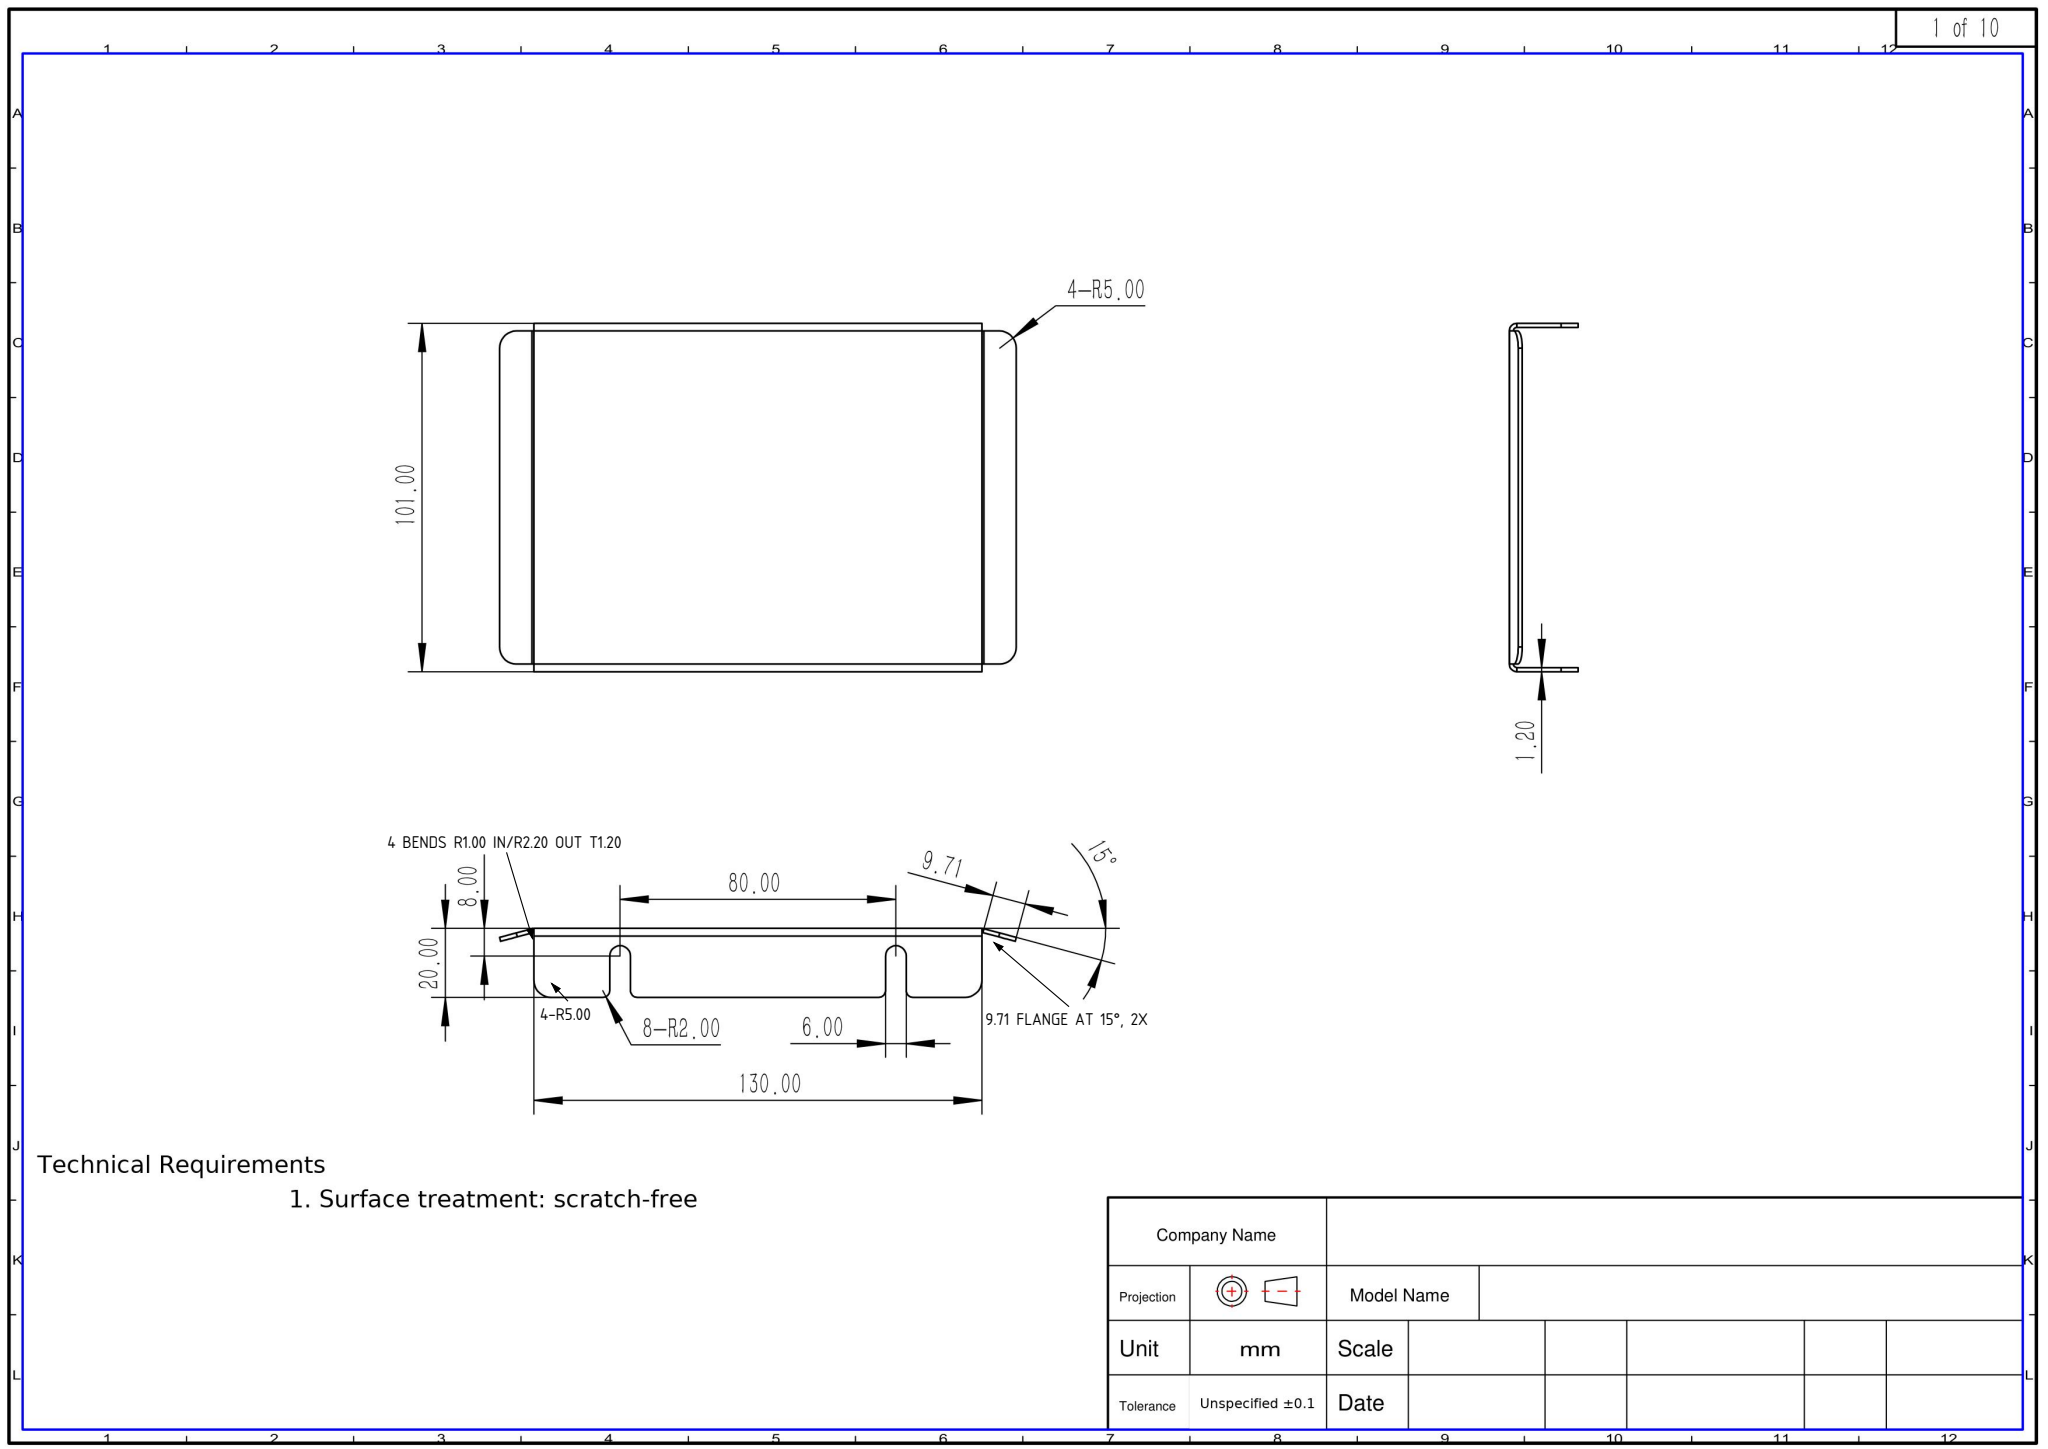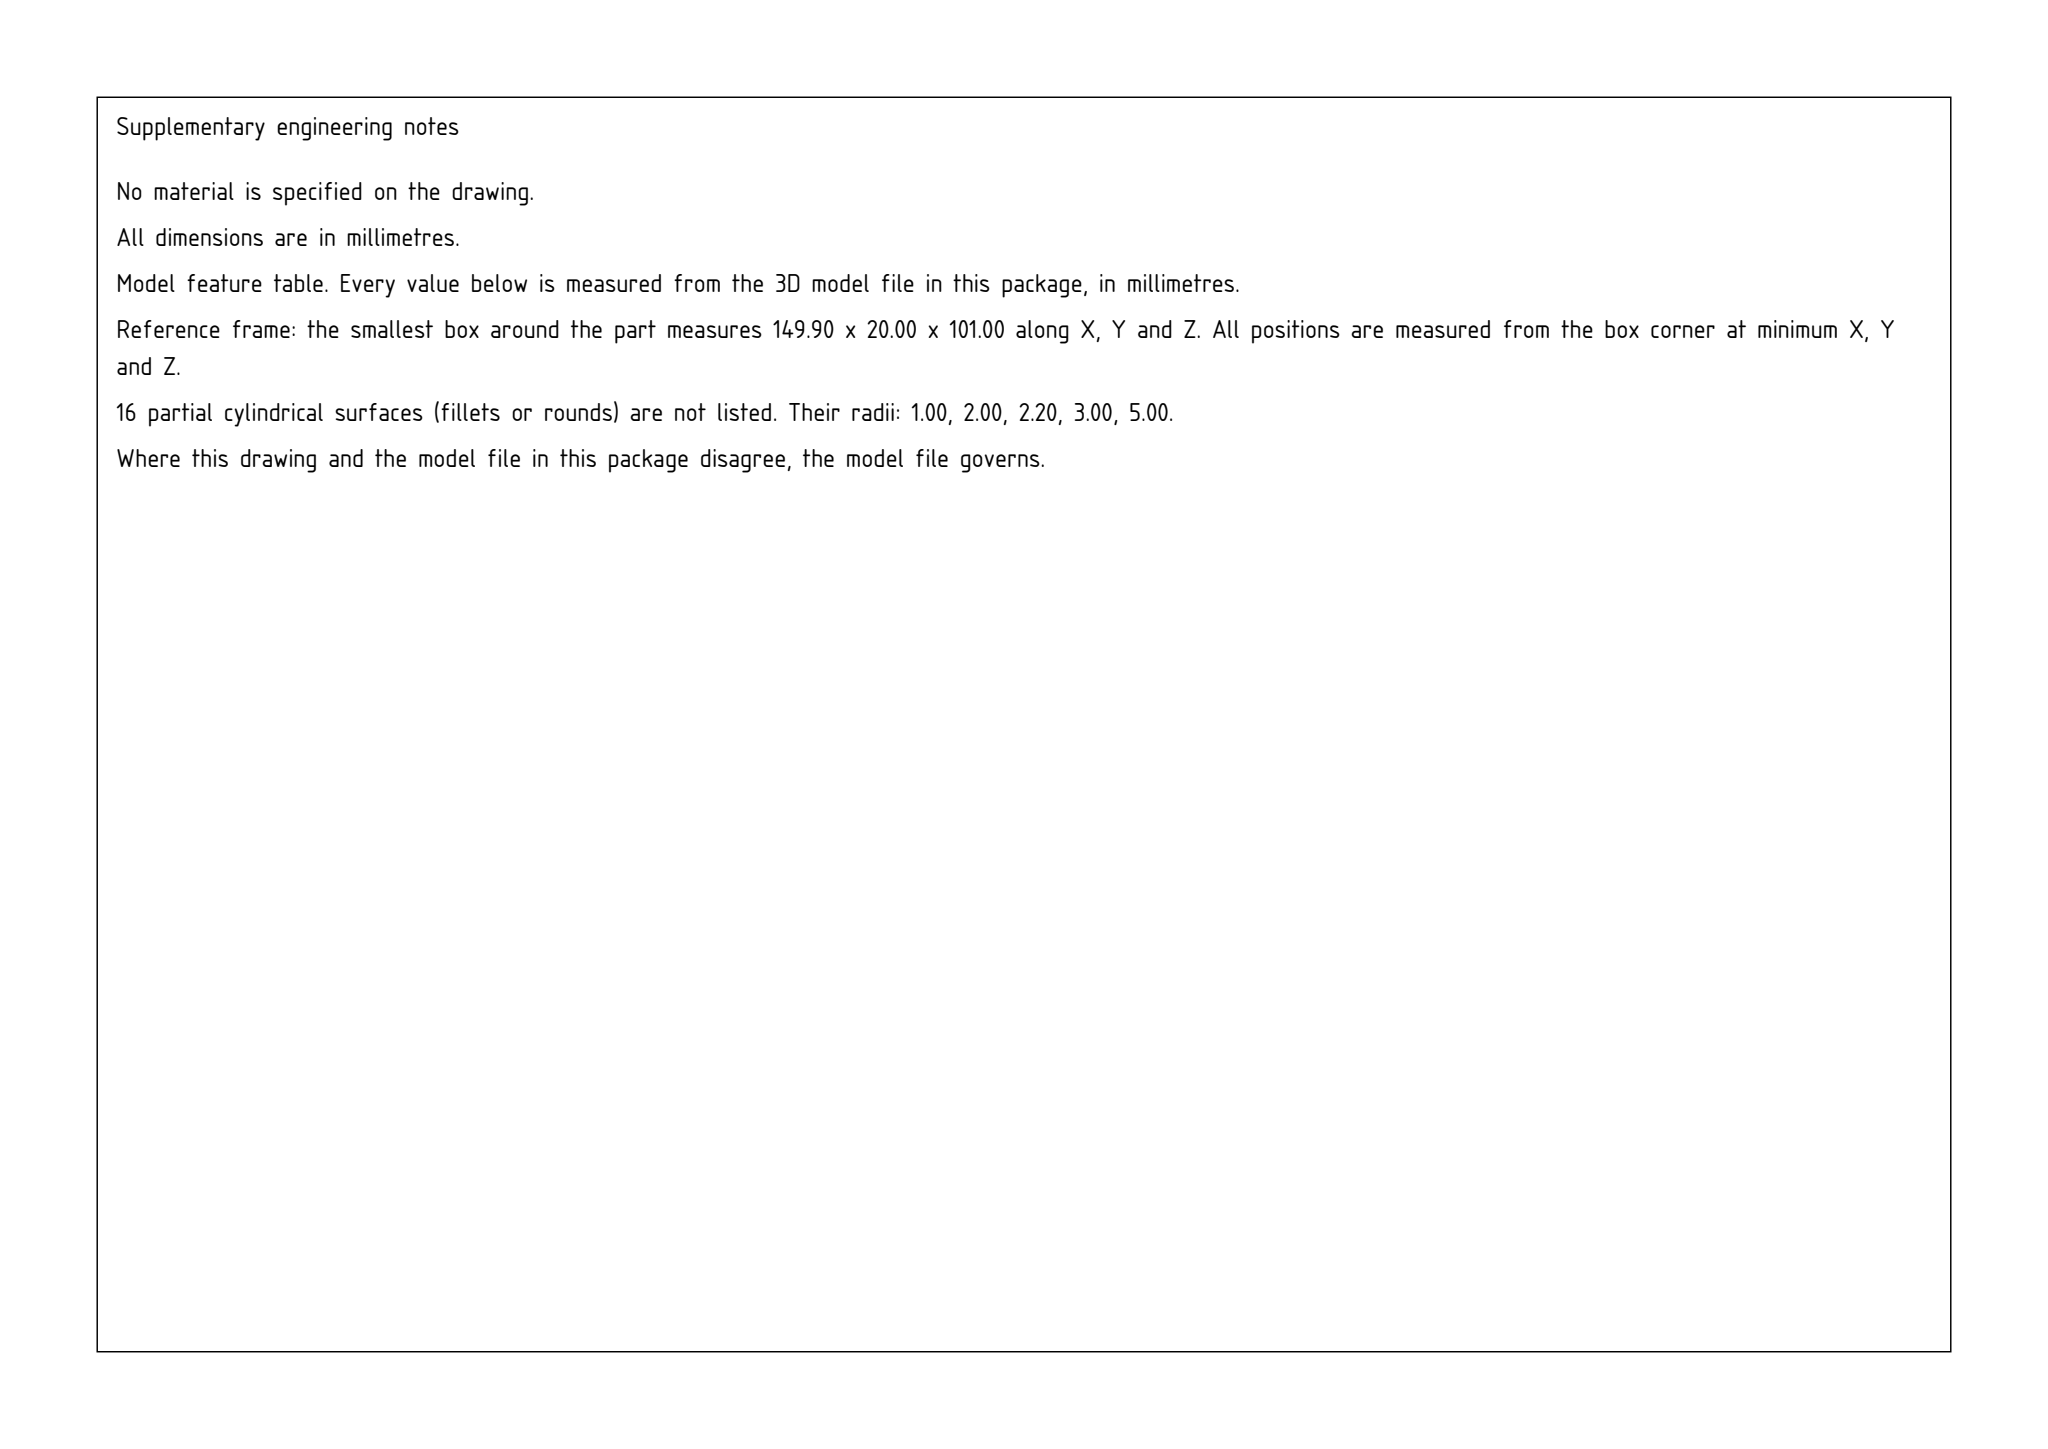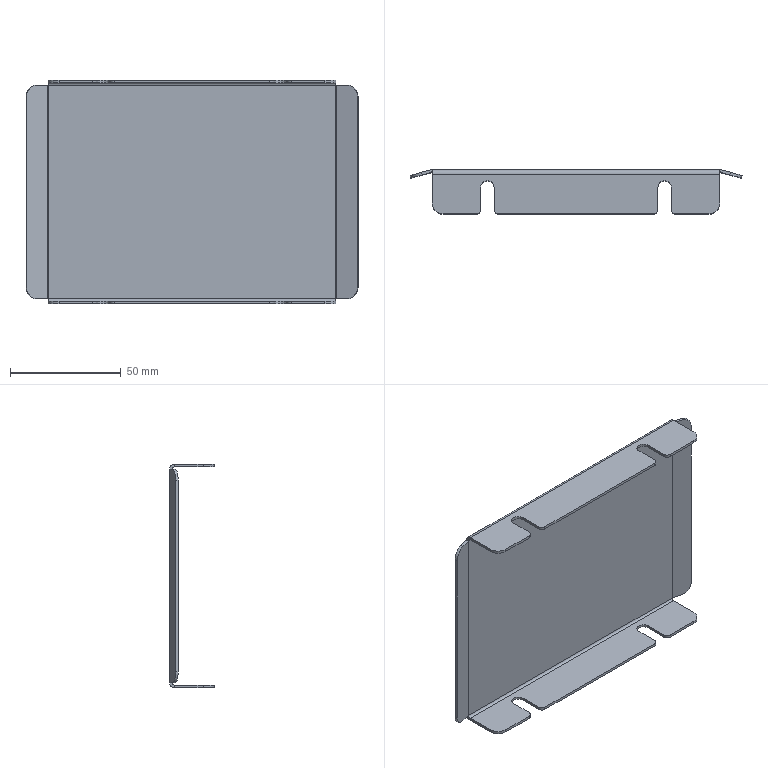Part | SolidWorks | mm | 1 solid | 70 faces | box 149.9 x 20 x 101 mm | volume 23283 mm3 | plane 42 | cylinder 28 | commonest cylinder face diameters 10 x8 4 x8 4.4 x4 2 x4 6 x4
Drawing notes:
15° FLANGE LEN 9.71 EA END, FRONT VIEW | from the solid: Inclined planes at 15° to X, size 9.4 x 2.5 -> length sqrt(9.4^2+2.5^2)=9.71; at x 0-9.4 and 140.2-149.6
ALL 4 BENDS: INSIDE R1.00, OUTSIDE R2.20, MATL THK 1.20 | from the solid: concave arcs dia 2.0 (R1.00) and convex arcs dia 4.4 (R2.20) at the two x-axis side-wall bends and two z-axis 15 deg flange bends; wall thk 20.0-18.8=1.2
FRONT VIEW: 4-R5.00 LOWER OUTER CORNERS OF SIDE WALLS (8-R5 TOT) | from the solid: convex arcs dia 10.0, axis z, centers (134.9,5.0) & (14.9,5.0), z 0-1.2 and 99.8-101.0, 90 deg each